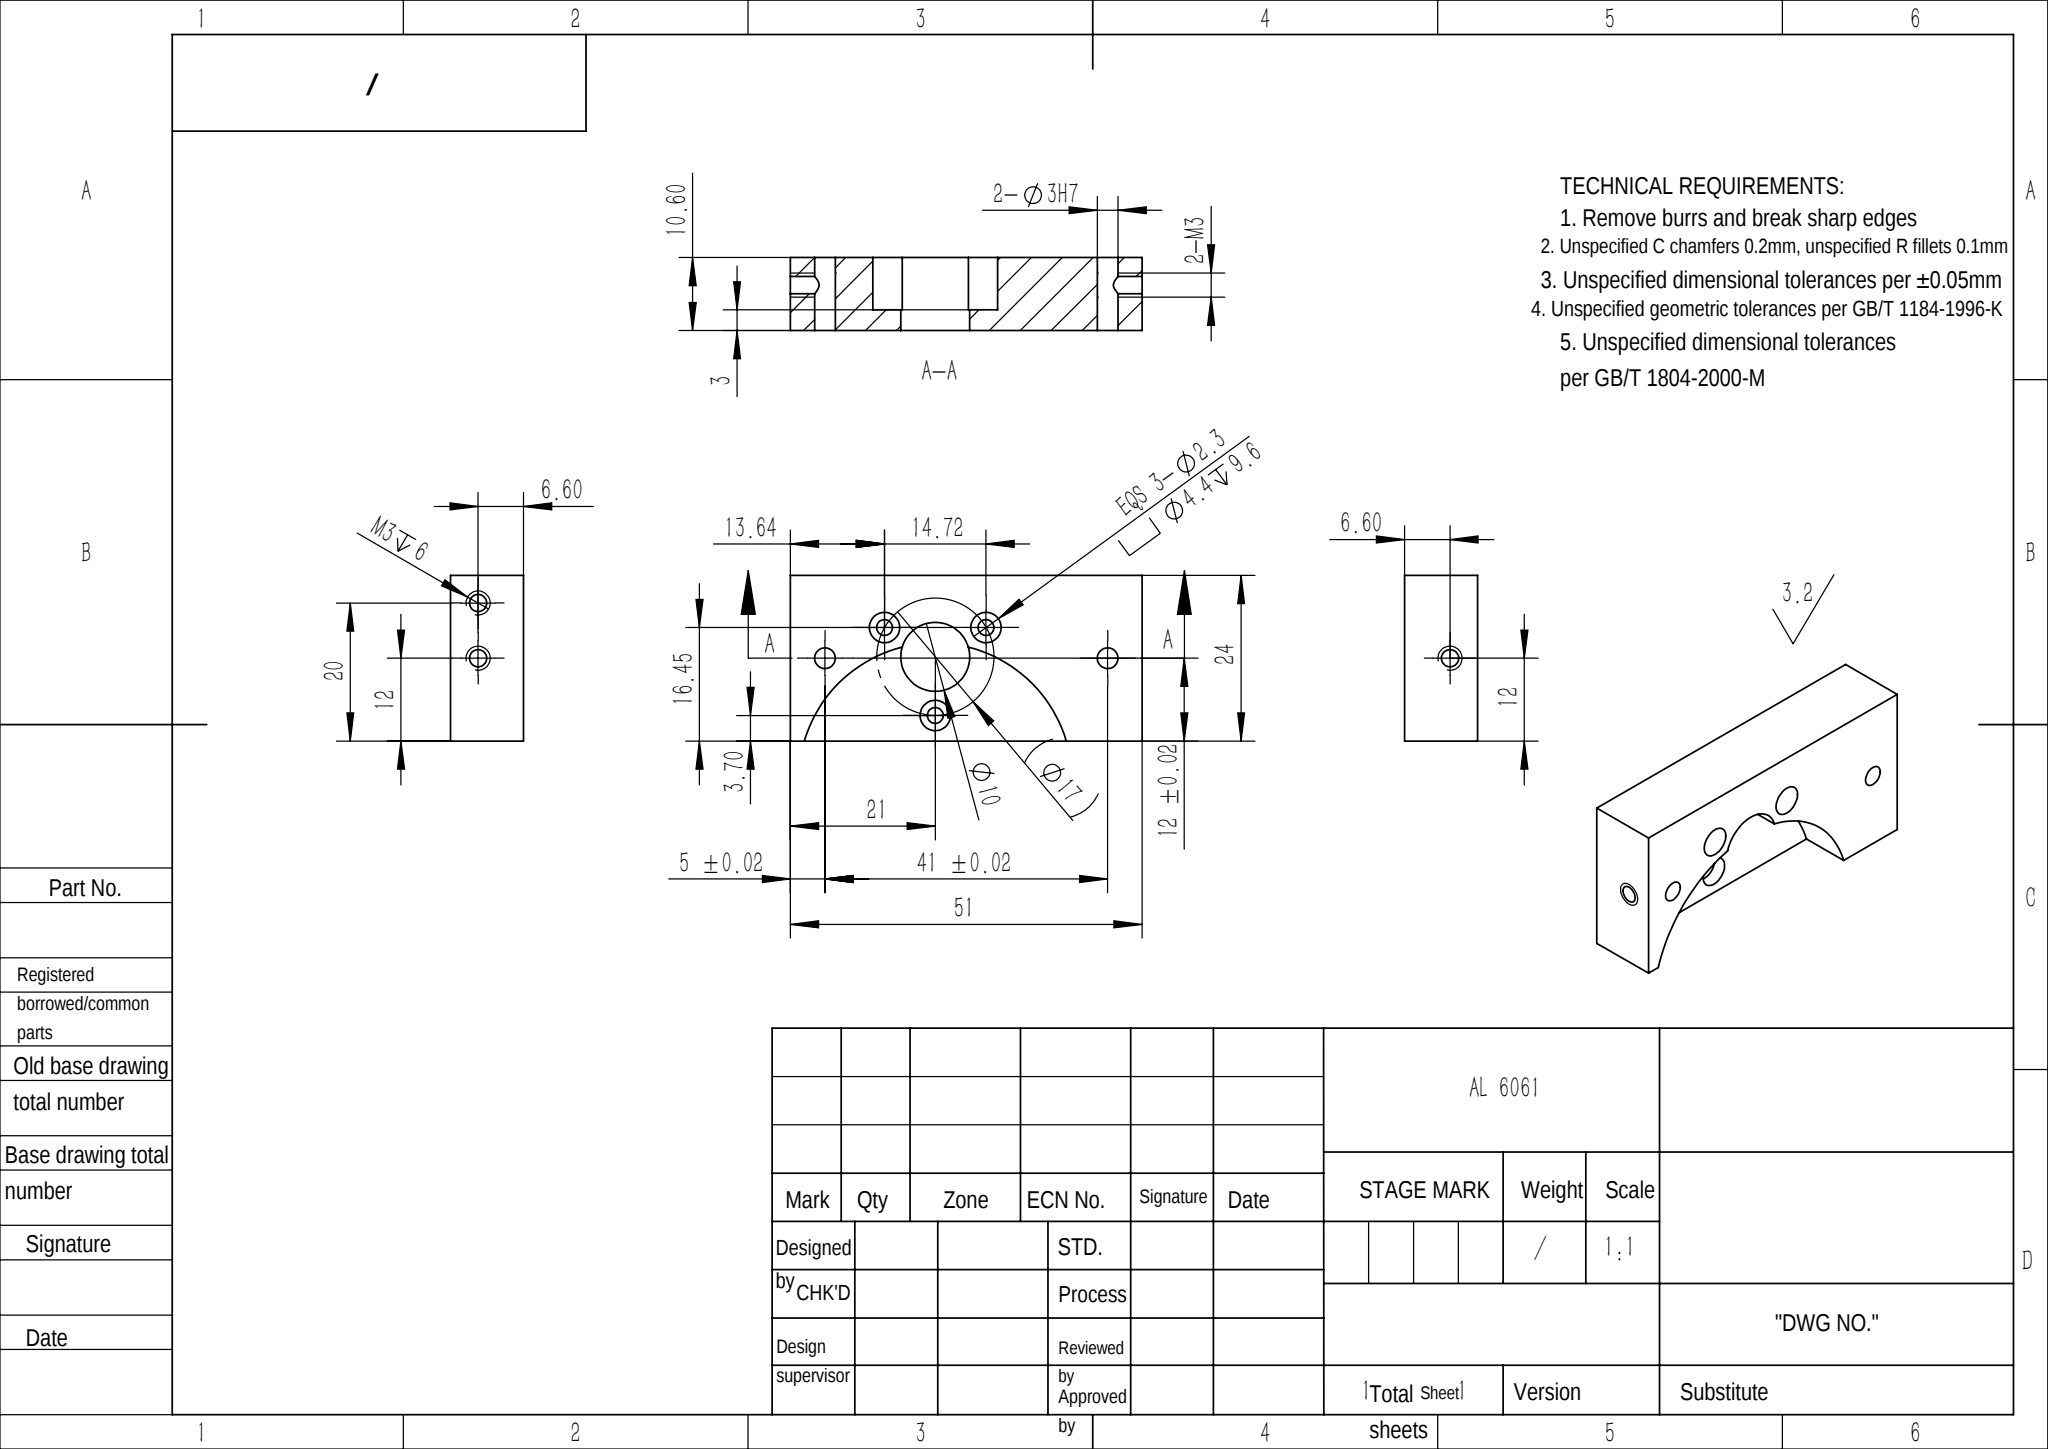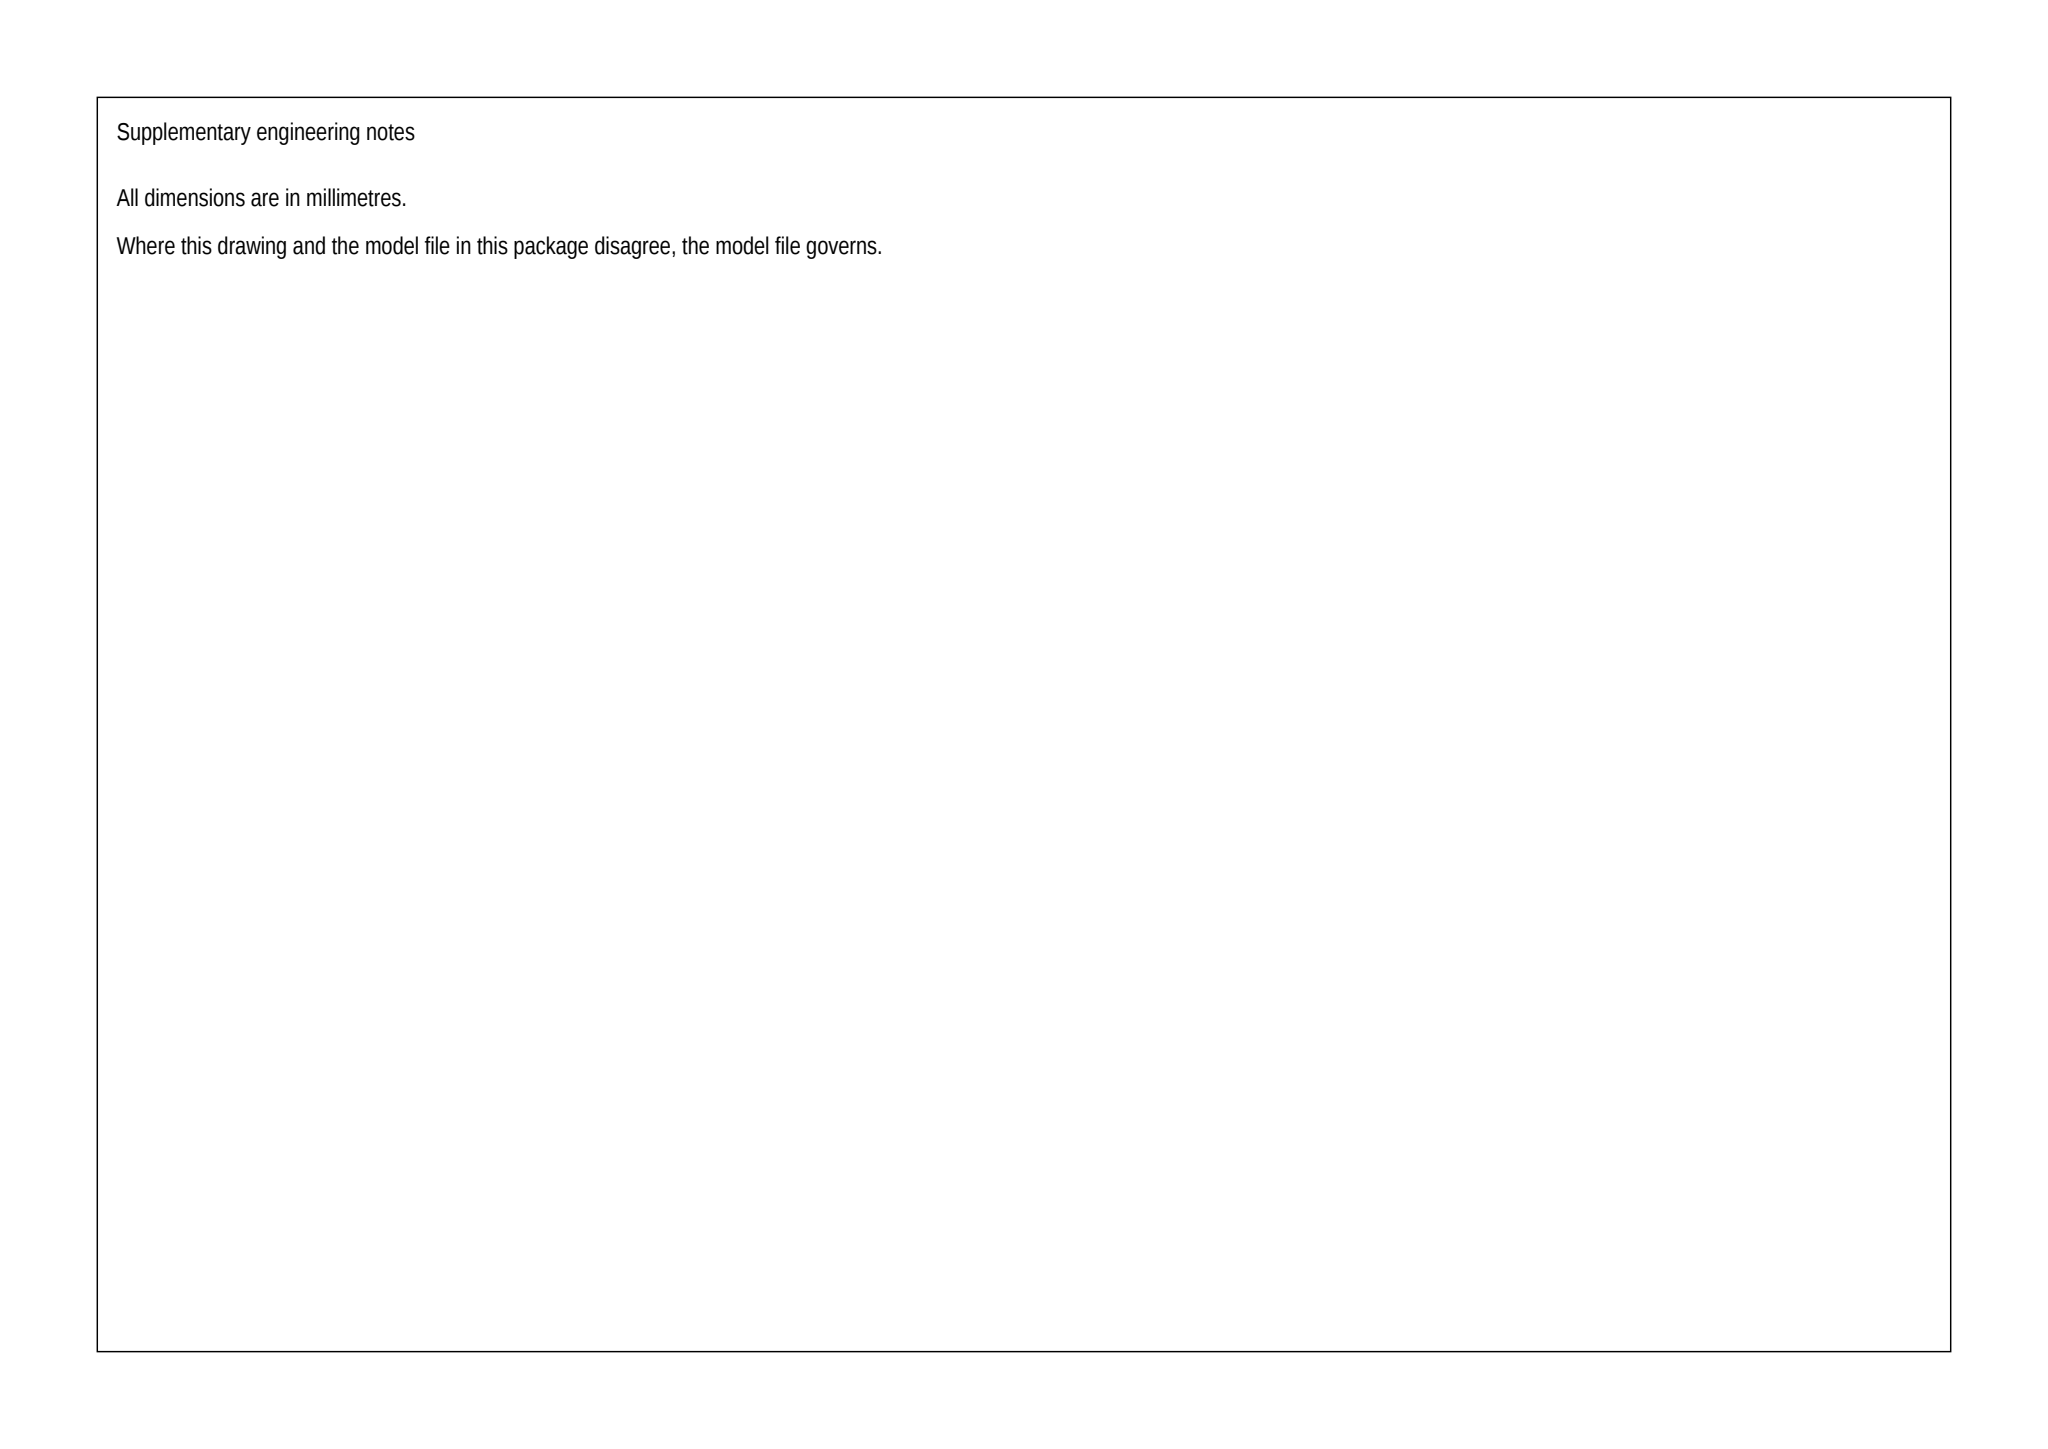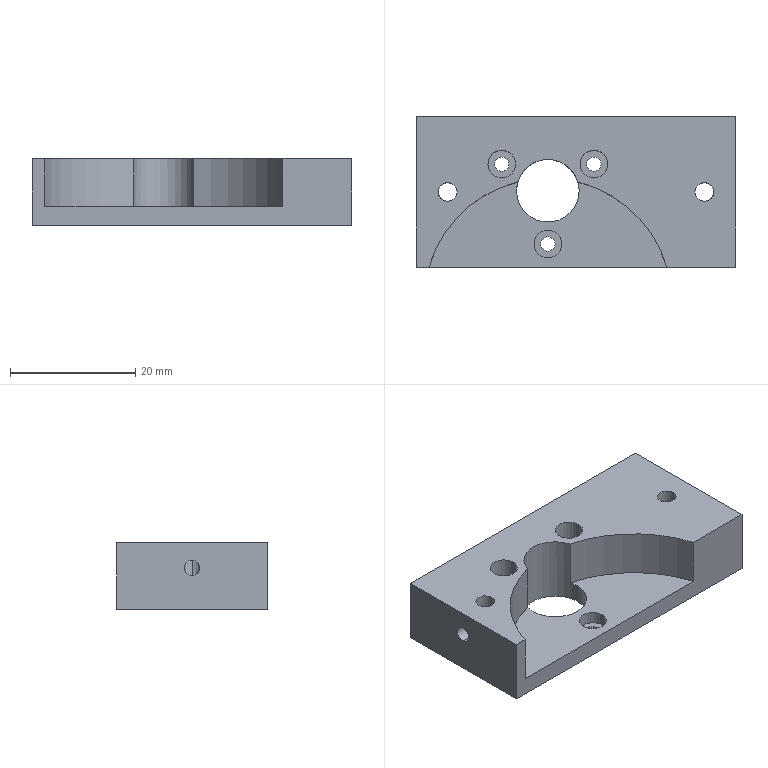Part | SolidWorks | mm | material AL 6061 | 1 solid | 37 faces | box 51 x 24 x 10.6 mm | volume 9004 mm3 | cylinder 26 | plane 11 | commonest cylinder face diameters 2.3 x6 4.4 x6 2.5 x6 3 x4 10 x2 39.633 x2